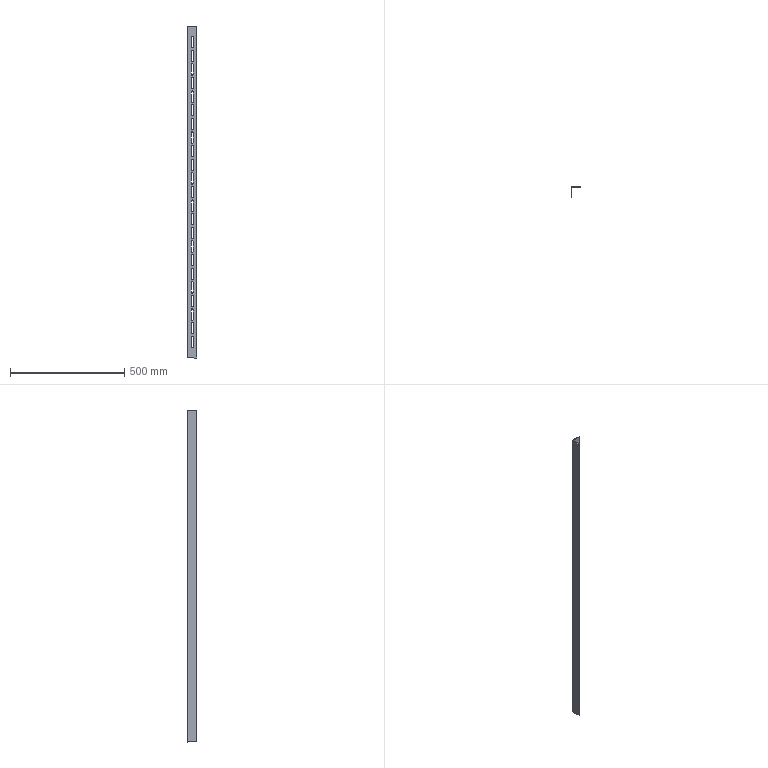Component | SolidWorks | Column-8 | 1 solid | 129 faces | volume 271464 mm3 | cylinder 71 | plane 58 | commonest cylinder face diameters 9 x69 1 x1 6 x1